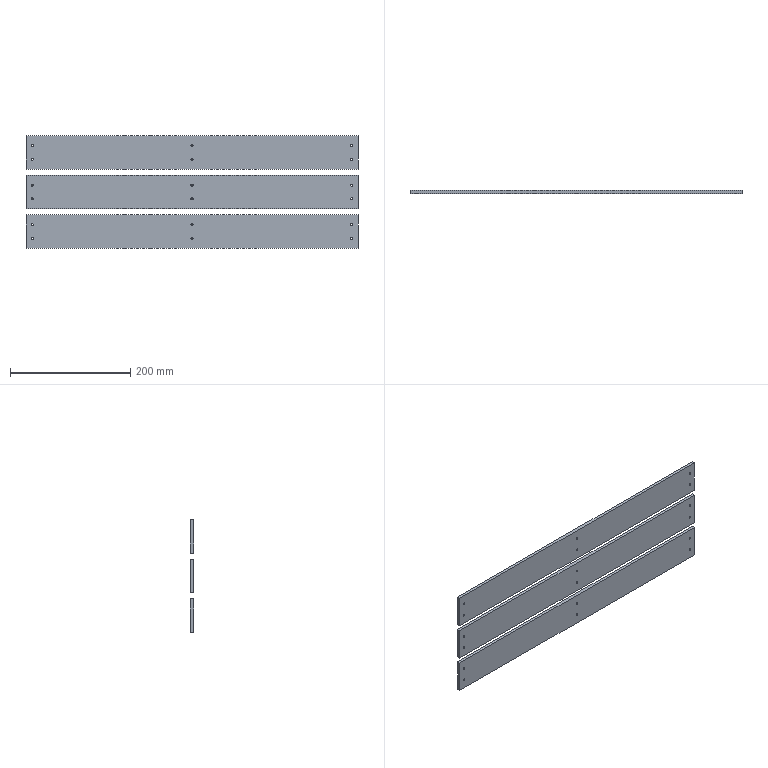CAM job | Mastercam | mm | 4 operations | part box 553 x 5 x 188
1. Contour (Ramp) | 4 - 4 平铣刀
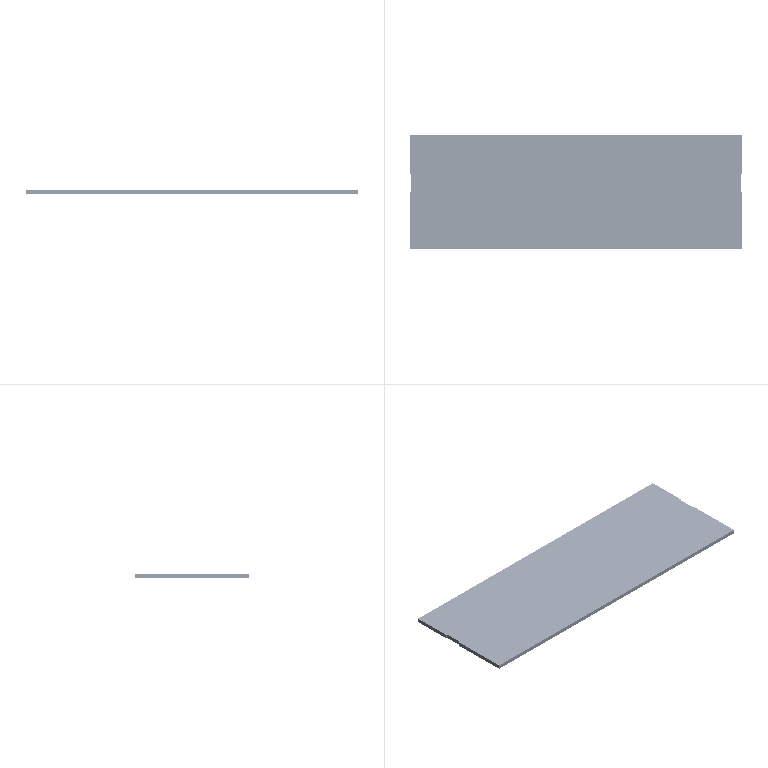2. Contour (2D) | 4 - 4 平铣刀
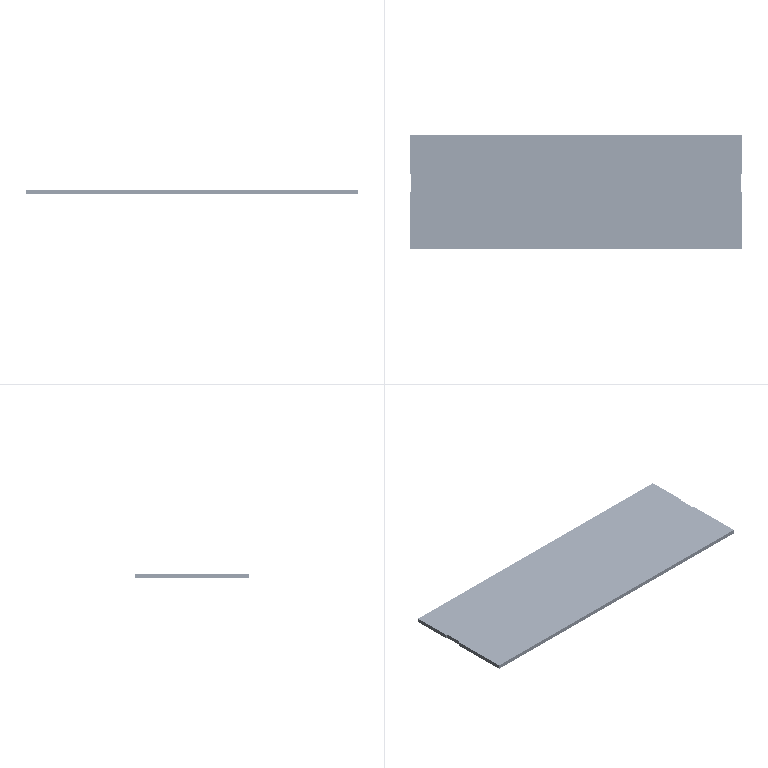3. Drill/Counterbore | 5 - 4 倒角刀
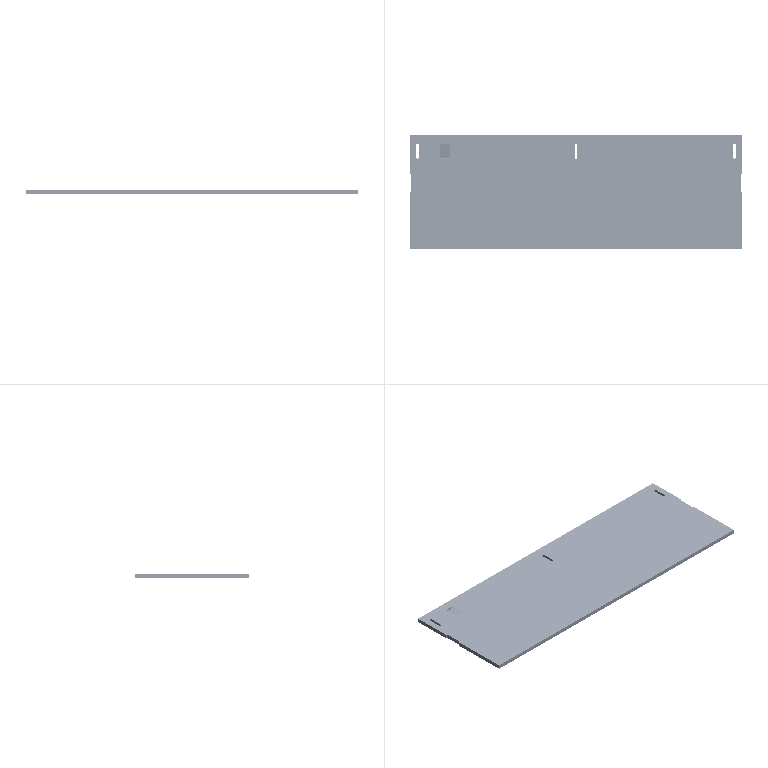4. Contour (2D chamfer) | 5 - 4 倒角刀